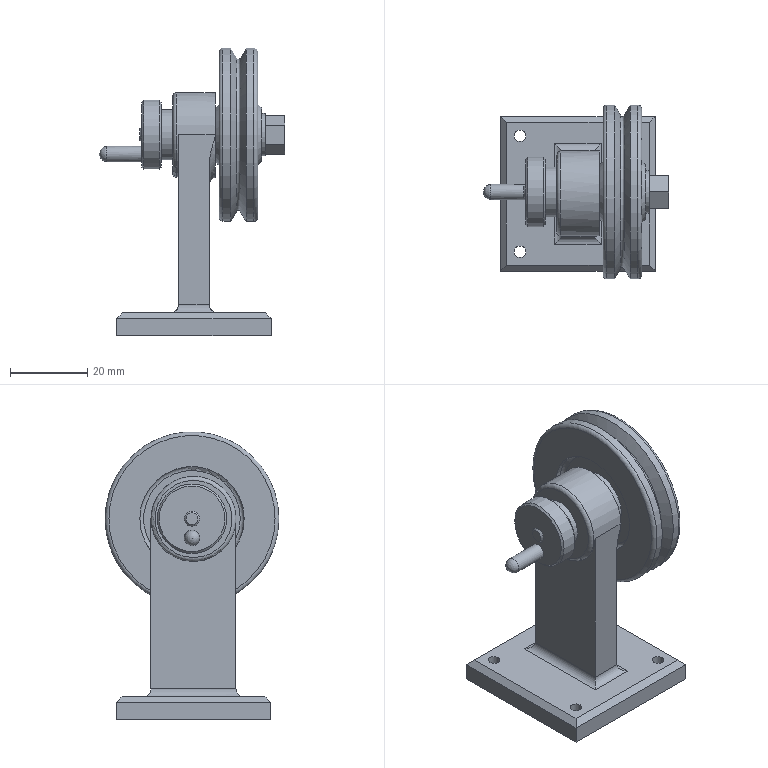Assembly | NX | mm | 9 component files | 9 solids | 110 faces | box 48 x 45 x 74.56 mm | volume 35202 mm3 | plane 53 | cylinder 37 | cone 11 | torus 7 | spline 1 | sphere 1 | commonest cylinder face diameters 3 x10 4 x8 8 x3 10 x2 27 x2 16 x2 45 x2 22 x1
Bill of materials:
unnamed part 1 | 1 |  | Disc-shaped grooved wheel with a V-profile groove around its outer edge, a raised central hub on both faces, and a central bore with one rectangular keyway notch.
unnamed part 2 | 1 |  | Thin flat ring (annular disc) with plain parallel faces and a concentric round through-hole.
unnamed part 3 | 1 |  | Hexagonal prism with a concentric round through-bore. The bore edge is chamfered or countersunk on the visible face.
unnamed part 4 | 1 |  | Stepped cylindrical pin. The main body is a larger-diameter cylinder with a closed-end elongated slot (slotted recess) on one side. A smaller pin with a chamfered end sticks out from one end, and a pin with a domed/rounded tip sticks out from the other, after a short neck step.
unnamed part 5 | 1 |  | Two-diameter stepped cylindrical pin. The larger section has a fully rounded (domed) end, and the smaller coaxial section has a chamfered flat end.
unnamed part 6 | 1 |  | Flanged cylindrical sleeve: a thin-walled tube with a larger-diameter flange at one end and a concentric through-bore.
unnamed part 7 | 1 |  | Thick round disc with chamfered outer edges on both faces and two round through-holes of different size. The larger hole is at the center and the smaller one is offset radially.
unnamed part 8 | 1 |  | Solid obround (stadium-shaped) prism: a straight extrusion with two flat parallel faces and fully rounded ends.
unnamed part 9 | 1 |  | Mounting bracket: a square base plate with chamfered top edges and four corner through-holes, plus a central upright rectangular post with a filleted root. The post ends in a rounded eye boss with a round through-hole that has a chamfered or counterbored entry.
Mates:
1. fix | Assy_Prac_Part_8 1 component
2. concentric | Assy_Prac_Part_2 1 edge | Assy_Prac_Part_8 1 edge
3. concentric | Assy_Prac_Part_3 1 edge | Assy_Prac_Part_2 1 edge
4. concentric | Assy_Prac_Part_7 1 edge | Assy_Prac_Part_3 1 edge
5. concentric | Assy_Prac_Part_1 1 edge | Assy_Prac_Part_3 1 edge
6. concentric | Assy_Prac_Part_9 1 edge | Assy_Prac_Part_8 1 edge
7. concentric | Assy_Prac_Part_5 1 edge | Assy_Prac_Part_9 1 edge
8. concentric | Assy_Prac_Part_4 1 edge | Assy_Prac_Part_5 1 edge